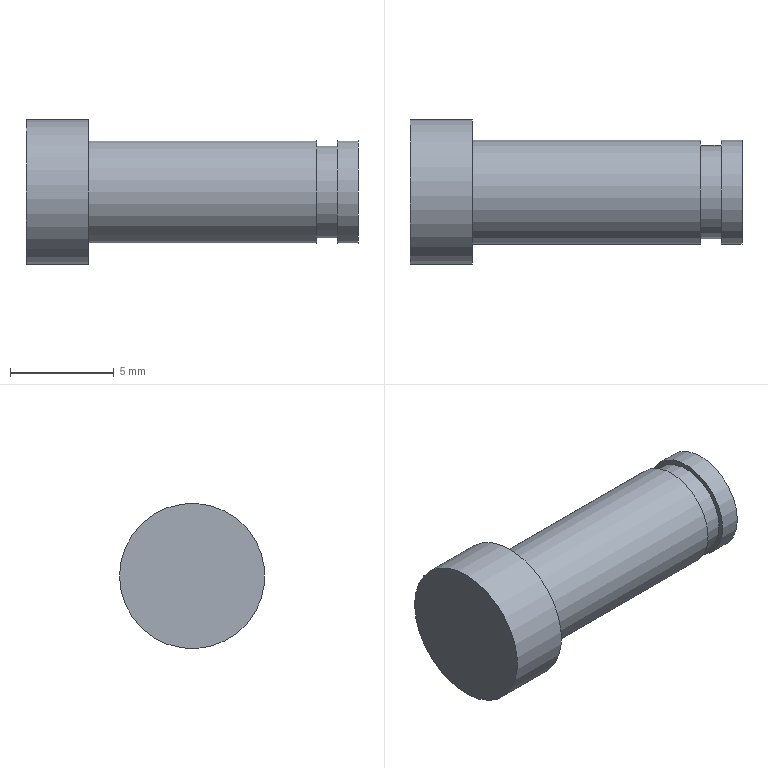Component | NX | PIN | 1 solid | 9 faces | box 16 x 7 x 7 mm | volume 367 mm3 | plane 5 | cylinder 4 | commonest cylinder face diameters 5 x2 7 x1 4.5 x1
STEP:
#1=CARTESIAN_POINT('',(0.,0.,0.));
#2=DIRECTION('',(0.,0.,1.));
#3=DIRECTION('',(1.,0.,0.));
#4=AXIS2_PLACEMENT_3D('',#1,#2,#3);
#5=CARTESIAN_POINT('',(-94.,4.863,83.));
#6=VERTEX_POINT('',#5);
#7=CARTESIAN_POINT('',(-94.,2.363,83.));
#8=DIRECTION('',(1.,0.,0.));
#9=DIRECTION('',(0.,1.,0.));
#10=AXIS2_PLACEMENT_3D('',#7,#8,#9);
#11=CIRCLE('',#10,2.5);
#12=CARTESIAN_POINT('',(-94.,2.363,83.));
#13=DIRECTION('',(1.,0.,0.));
#14=DIRECTION('',(0.,1.,0.));
#15=AXIS2_PLACEMENT_3D('',#12,#13,#14);
#16=PLANE('',#15);
#17=CARTESIAN_POINT('',(0.,0.));
#18=DIRECTION('',(1.,0.));
#19=AXIS2_PLACEMENT_2D('',#17,#18);
#20=CIRCLE('',#19,2.5);
#21=(GEOMETRIC_REPRESENTATION_CONTEXT(2)PARAMETRIC_REPRESENTATION_CONTEXT()REPRESENTATION_CONTEXT('',''));
#22=DEFINITIONAL_REPRESENTATION('',(#20),#21);
#23=PCURVE('',#16,#22);
#24=CARTESIAN_POINT('',(-94.,2.363,83.));
#25=DIRECTION('',(1.,0.,0.));
#26=DIRECTION('',(0.,1.,0.));
#27=AXIS2_PLACEMENT_3D('',#24,#25,#26);
#28=CYLINDRICAL_SURFACE('',#27,2.5);
#29=CARTESIAN_POINT('',(0.,0.));
#30=DIRECTION('',(1.,0.));
#31=VECTOR('',#30,1.);
#32=LINE('',#29,#31);
#33=(GEOMETRIC_REPRESENTATION_CONTEXT(2)PARAMETRIC_REPRESENTATION_CONTEXT()REPRESENTATION_CONTEXT('',''));
#34=DEFINITIONAL_REPRESENTATION('',(#32),#33);
#35=PCURVE('',#28,#34);
#36=SURFACE_CURVE('',#11,(#23,#35),.PCURVE_S1.);
#37=EDGE_CURVE('',#6,#6,#36,.T.);
#38=ORIENTED_EDGE('',*,*,#37,.F.);
#39=EDGE_LOOP('',(#38));
#40=FACE_BOUND('',#39,.T.);
#41=CARTESIAN_POINT('',(-94.,5.863,83.));
#42=VERTEX_POINT('',#41);
#43=CARTESIAN_POINT('',(-94.,2.363,83.));
#44=DIRECTION('',(-1.,0.,0.));
#45=DIRECTION('',(0.,1.,0.));
#46=AXIS2_PLACEMENT_3D('',#43,#44,#45);
#47=CIRCLE('',#46,3.5);
#48=CARTESIAN_POINT('',(3.5,0.));
#49=CARTESIAN_POINT('',(3.5,-6.062));
#50=CARTESIAN_POINT('',(-1.75,-3.031));
#51=CARTESIAN_POINT('',(-7.,-0.));
#52=CARTESIAN_POINT('',(-1.75,3.031));
#53=CARTESIAN_POINT('',(3.5,6.062));
#54=CARTESIAN_POINT('',(3.5,0.));
#55=(BOUNDED_CURVE()B_SPLINE_CURVE(2,(#48,#49,#50,#51,#52,#53,#54),.UNSPECIFIED.,.T.,.F.)B_SPLINE_CURVE_WITH_KNOTS((1,2,2,2,2,1),(-2.094,0.,2.094,4.189,6.283,8.378),.UNSPECIFIED.)CURVE()GEOMETRIC_REPRESENTATION_ITEM()RATIONAL_B_SPLINE_CURVE((1.,0.5,1.,0.5,1.,0.5,1.))REPRESENTATION_ITEM(''));
#56=(GEOMETRIC_REPRESENTATION_CONTEXT(2)PARAMETRIC_REPRESENTATION_CONTEXT()REPRESENTATION_CONTEXT('',''));
#57=DEFINITIONAL_REPRESENTATION('',(#55),#56);
#58=PCURVE('',#16,#57);
#59=CARTESIAN_POINT('',(-97.,2.363,83.));
#60=DIRECTION('',(1.,0.,0.));
#61=DIRECTION('',(0.,1.,0.));
#62=AXIS2_PLACEMENT_3D('',#59,#60,#61);
#63=CYLINDRICAL_SURFACE('',#62,3.5);
#64=CARTESIAN_POINT('',(6.283,3.));
#65=DIRECTION('',(-1.,0.));
#66=VECTOR('',#65,1.);
#67=LINE('',#64,#66);
#68=(GEOMETRIC_REPRESENTATION_CONTEXT(2)PARAMETRIC_REPRESENTATION_CONTEXT()REPRESENTATION_CONTEXT('',''));
#69=DEFINITIONAL_REPRESENTATION('',(#67),#68);
#70=PCURVE('',#63,#69);
#71=SURFACE_CURVE('',#47,(#58,#70),.PCURVE_S1.);
#72=EDGE_CURVE('',#42,#42,#71,.T.);
#73=ORIENTED_EDGE('',*,*,#72,.F.);
#74=EDGE_LOOP('',(#73));
#75=FACE_BOUND('',#74,.T.);
#76=ADVANCED_FACE('',(#40,#75),#16,.T.);
#77=CARTESIAN_POINT('',(-97.,5.863,83.));
#78=VERTEX_POINT('',#77);
#79=CARTESIAN_POINT('',(-97.,2.363,83.));
#80=DIRECTION('',(1.,0.,0.));
#81=DIRECTION('',(0.,1.,0.));
#82=AXIS2_PLACEMENT_3D('',#79,#80,#81);
#83=CIRCLE('',#82,3.5);
#84=CARTESIAN_POINT('',(-97.,2.363,83.));
#85=DIRECTION('',(-1.,0.,0.));
#86=DIRECTION('',(0.,-1.,0.));
#87=AXIS2_PLACEMENT_3D('',#84,#85,#86);
#88=PLANE('',#87);
#89=CARTESIAN_POINT('',(-3.5,0.));
#90=CARTESIAN_POINT('',(-3.5,6.062));
#91=CARTESIAN_POINT('',(1.75,3.031));
#92=CARTESIAN_POINT('',(7.,0.));
#93=CARTESIAN_POINT('',(1.75,-3.031));
#94=CARTESIAN_POINT('',(-3.5,-6.062));
#95=CARTESIAN_POINT('',(-3.5,0.));
#96=(BOUNDED_CURVE()B_SPLINE_CURVE(2,(#89,#90,#91,#92,#93,#94,#95),.UNSPECIFIED.,.T.,.F.)B_SPLINE_CURVE_WITH_KNOTS((1,2,2,2,2,1),(-2.094,0.,2.094,4.189,6.283,8.378),.UNSPECIFIED.)CURVE()GEOMETRIC_REPRESENTATION_ITEM()RATIONAL_B_SPLINE_CURVE((1.,0.5,1.,0.5,1.,0.5,1.))REPRESENTATION_ITEM(''));
#97=(GEOMETRIC_REPRESENTATION_CONTEXT(2)PARAMETRIC_REPRESENTATION_CONTEXT()REPRESENTATION_CONTEXT('',''));
#98=DEFINITIONAL_REPRESENTATION('',(#96),#97);
#99=PCURVE('',#88,#98);
#100=CARTESIAN_POINT('',(0.,0.));
#101=DIRECTION('',(1.,0.));
#102=VECTOR('',#101,1.);
#103=LINE('',#100,#102);
#104=(GEOMETRIC_REPRESENTATION_CONTEXT(2)PARAMETRIC_REPRESENTATION_CONTEXT()REPRESENTATION_CONTEXT('',''));
#105=DEFINITIONAL_REPRESENTATION('',(#103),#104);
#106=PCURVE('',#63,#105);
#107=SURFACE_CURVE('',#83,(#99,#106),.PCURVE_S1.);
#108=EDGE_CURVE('',#78,#78,#107,.T.);
#109=ORIENTED_EDGE('',*,*,#108,.F.);
#110=EDGE_LOOP('',(#109));
#111=FACE_BOUND('',#110,.T.);
#112=ADVANCED_FACE('',(#111),#88,.T.);
#113=ORIENTED_EDGE('',*,*,#72,.T.);
#114=CARTESIAN_POINT('',(-97.,5.863,83.));
#115=CARTESIAN_POINT('',(-94.,5.863,83.));
#116=B_SPLINE_CURVE_WITH_KNOTS('',1,(#114,#115),.UNSPECIFIED.,.F.,.F.,(2,2),(0.,3.),.PIECEWISE_BEZIER_KNOTS.);
#117=CARTESIAN_POINT('',(0.,0.));
#118=DIRECTION('',(0.,1.));
#119=VECTOR('',#118,1.);
#120=LINE('',#117,#119);
#121=(GEOMETRIC_REPRESENTATION_CONTEXT(2)PARAMETRIC_REPRESENTATION_CONTEXT()REPRESENTATION_CONTEXT('',''));
#122=DEFINITIONAL_REPRESENTATION('',(#120),#121);
#123=PCURVE('',#63,#122);
#124=CARTESIAN_POINT('',(6.283,0.));
#125=DIRECTION('',(0.,1.));
#126=VECTOR('',#125,1.);
#127=LINE('',#124,#126);
#128=(GEOMETRIC_REPRESENTATION_CONTEXT(2)PARAMETRIC_REPRESENTATION_CONTEXT()REPRESENTATION_CONTEXT('',''));
#129=DEFINITIONAL_REPRESENTATION('',(#127),#128);
#130=PCURVE('',#63,#129);
#131=SEAM_CURVE('',#116,(#123,#130),.PCURVE_S1.);
#132=EDGE_CURVE('',#78,#42,#131,.T.);
#133=ORIENTED_EDGE('',*,*,#132,.F.);
#134=ORIENTED_EDGE('',*,*,#108,.T.);
#135=ORIENTED_EDGE('',*,*,#132,.T.);
#136=EDGE_LOOP('',(#113,#133,#134,#135));
#137=FACE_BOUND('',#136,.T.);
#138=ADVANCED_FACE('',(#137),#63,.T.);
#139=CARTESIAN_POINT('',(-83.,4.613,83.));
#140=VERTEX_POINT('',#139);
#141=CARTESIAN_POINT('',(-83.,2.363,83.));
#142=DIRECTION('',(1.,0.,0.));
#143=DIRECTION('',(0.,1.,0.));
#144=AXIS2_PLACEMENT_3D('',#141,#142,#143);
#145=CIRCLE('',#144,2.25);
#146=CARTESIAN_POINT('',(-83.,2.363,83.));
#147=DIRECTION('',(1.,0.,0.));
#148=DIRECTION('',(0.,1.,0.));
#149=AXIS2_PLACEMENT_3D('',#146,#147,#148);
#150=PLANE('',#149);
#151=CARTESIAN_POINT('',(0.,0.));
#152=DIRECTION('',(1.,0.));
#153=AXIS2_PLACEMENT_2D('',#151,#152);
#154=CIRCLE('',#153,2.25);
#155=(GEOMETRIC_REPRESENTATION_CONTEXT(2)PARAMETRIC_REPRESENTATION_CONTEXT()REPRESENTATION_CONTEXT('',''));
#156=DEFINITIONAL_REPRESENTATION('',(#154),#155);
#157=PCURVE('',#150,#156);
#158=CARTESIAN_POINT('',(-83.,2.363,83.));
#159=DIRECTION('',(1.,0.,0.));
#160=DIRECTION('',(0.,1.,0.));
#161=AXIS2_PLACEMENT_3D('',#158,#159,#160);
#162=CYLINDRICAL_SURFACE('',#161,2.25);
#163=CARTESIAN_POINT('',(0.,0.));
#164=DIRECTION('',(1.,0.));
#165=VECTOR('',#164,1.);
#166=LINE('',#163,#165);
#167=(GEOMETRIC_REPRESENTATION_CONTEXT(2)PARAMETRIC_REPRESENTATION_CONTEXT()REPRESENTATION_CONTEXT('',''));
#168=DEFINITIONAL_REPRESENTATION('',(#166),#167);
#169=PCURVE('',#162,#168);
#170=SURFACE_CURVE('',#145,(#157,#169),.PCURVE_S1.);
#171=EDGE_CURVE('',#140,#140,#170,.T.);
#172=ORIENTED_EDGE('',*,*,#171,.F.);
#173=EDGE_LOOP('',(#172));
#174=FACE_BOUND('',#173,.T.);
#175=CARTESIAN_POINT('',(-83.,4.863,83.));
#176=VERTEX_POINT('',#175);
#177=CARTESIAN_POINT('',(-83.,2.363,83.));
#178=DIRECTION('',(1.,0.,0.));
#179=DIRECTION('',(0.,1.,0.));
#180=AXIS2_PLACEMENT_3D('',#177,#178,#179);
#181=CIRCLE('',#180,2.5);
#182=CARTESIAN_POINT('',(0.,0.));
#183=DIRECTION('',(1.,0.));
#184=AXIS2_PLACEMENT_2D('',#182,#183);
#185=CIRCLE('',#184,2.5);
#186=(GEOMETRIC_REPRESENTATION_CONTEXT(2)PARAMETRIC_REPRESENTATION_CONTEXT()REPRESENTATION_CONTEXT('',''));
#187=DEFINITIONAL_REPRESENTATION('',(#185),#186);
#188=PCURVE('',#150,#187);
#189=CARTESIAN_POINT('',(0.,11.));
#190=DIRECTION('',(1.,0.));
#191=VECTOR('',#190,1.);
#192=LINE('',#189,#191);
#193=(GEOMETRIC_REPRESENTATION_CONTEXT(2)PARAMETRIC_REPRESENTATION_CONTEXT()REPRESENTATION_CONTEXT('',''));
#194=DEFINITIONAL_REPRESENTATION('',(#192),#193);
#195=PCURVE('',#28,#194);
#196=SURFACE_CURVE('',#181,(#188,#195),.PCURVE_S1.);
#197=EDGE_CURVE('',#176,#176,#196,.T.);
#198=ORIENTED_EDGE('',*,*,#197,.T.);
#199=EDGE_LOOP('',(#198));
#200=FACE_BOUND('',#199,.T.);
#201=ADVANCED_FACE('',(#174,#200),#150,.T.);
#202=ORIENTED_EDGE('',*,*,#197,.F.);
#203=CARTESIAN_POINT('',(-94.,4.863,83.));
#204=CARTESIAN_POINT('',(-83.,4.863,83.));
#205=B_SPLINE_CURVE_WITH_KNOTS('',1,(#203,#204),.UNSPECIFIED.,.F.,.F.,(2,2),(0.,11.),.PIECEWISE_BEZIER_KNOTS.);
#206=CARTESIAN_POINT('',(0.,0.));
#207=DIRECTION('',(0.,1.));
#208=VECTOR('',#207,1.);
#209=LINE('',#206,#208);
#210=(GEOMETRIC_REPRESENTATION_CONTEXT(2)PARAMETRIC_REPRESENTATION_CONTEXT()REPRESENTATION_CONTEXT('',''));
#211=DEFINITIONAL_REPRESENTATION('',(#209),#210);
#212=PCURVE('',#28,#211);
#213=CARTESIAN_POINT('',(6.283,0.));
#214=DIRECTION('',(0.,1.));
#215=VECTOR('',#214,1.);
#216=LINE('',#213,#215);
#217=(GEOMETRIC_REPRESENTATION_CONTEXT(2)PARAMETRIC_REPRESENTATION_CONTEXT()REPRESENTATION_CONTEXT('',''));
#218=DEFINITIONAL_REPRESENTATION('',(#216),#217);
#219=PCURVE('',#28,#218);
#220=SEAM_CURVE('',#205,(#212,#219),.PCURVE_S1.);
#221=EDGE_CURVE('',#6,#176,#220,.T.);
#222=ORIENTED_EDGE('',*,*,#221,.F.);
#223=ORIENTED_EDGE('',*,*,#37,.T.);
#224=ORIENTED_EDGE('',*,*,#221,.T.);
#225=EDGE_LOOP('',(#202,#222,#223,#224));
#226=FACE_BOUND('',#225,.T.);
#227=ADVANCED_FACE('',(#226),#28,.T.);
#228=CARTESIAN_POINT('',(-82.,4.613,83.));
#229=VERTEX_POINT('',#228);
#230=CARTESIAN_POINT('',(-82.,2.363,83.));
#231=DIRECTION('',(1.,0.,0.));
#232=DIRECTION('',(0.,1.,0.));
#233=AXIS2_PLACEMENT_3D('',#230,#231,#232);
#234=CIRCLE('',#233,2.25);
#235=CARTESIAN_POINT('',(0.,1.));
#236=DIRECTION('',(1.,0.));
#237=VECTOR('',#236,1.);
#238=LINE('',#235,#237);
#239=(GEOMETRIC_REPRESENTATION_CONTEXT(2)PARAMETRIC_REPRESENTATION_CONTEXT()REPRESENTATION_CONTEXT('',''));
#240=DEFINITIONAL_REPRESENTATION('',(#238),#239);
#241=PCURVE('',#162,#240);
#242=CARTESIAN_POINT('',(-82.,2.363,83.));
#243=DIRECTION('',(-1.,0.,0.));
#244=DIRECTION('',(0.,-1.,0.));
#245=AXIS2_PLACEMENT_3D('',#242,#243,#244);
#246=PLANE('',#245);
#247=CARTESIAN_POINT('',(-2.25,0.));
#248=CARTESIAN_POINT('',(-2.25,3.897));
#249=CARTESIAN_POINT('',(1.125,1.949));
#250=CARTESIAN_POINT('',(4.5,0.));
#251=CARTESIAN_POINT('',(1.125,-1.949));
#252=CARTESIAN_POINT('',(-2.25,-3.897));
#253=CARTESIAN_POINT('',(-2.25,0.));
#254=(BOUNDED_CURVE()B_SPLINE_CURVE(2,(#247,#248,#249,#250,#251,#252,#253),.UNSPECIFIED.,.T.,.F.)B_SPLINE_CURVE_WITH_KNOTS((1,2,2,2,2,1),(-2.094,0.,2.094,4.189,6.283,8.378),.UNSPECIFIED.)CURVE()GEOMETRIC_REPRESENTATION_ITEM()RATIONAL_B_SPLINE_CURVE((1.,0.5,1.,0.5,1.,0.5,1.))REPRESENTATION_ITEM(''));
#255=(GEOMETRIC_REPRESENTATION_CONTEXT(2)PARAMETRIC_REPRESENTATION_CONTEXT()REPRESENTATION_CONTEXT('',''));
#256=DEFINITIONAL_REPRESENTATION('',(#254),#255);
#257=PCURVE('',#246,#256);
#258=SURFACE_CURVE('',#234,(#241,#257),.PCURVE_S1.);
#259=EDGE_CURVE('',#229,#229,#258,.T.);
#260=ORIENTED_EDGE('',*,*,#259,.F.);
#261=CARTESIAN_POINT('',(-83.,4.613,83.));
#262=CARTESIAN_POINT('',(-82.,4.613,83.));
#263=B_SPLINE_CURVE_WITH_KNOTS('',1,(#261,#262),.UNSPECIFIED.,.F.,.F.,(2,2),(0.,1.),.PIECEWISE_BEZIER_KNOTS.);
#264=CARTESIAN_POINT('',(0.,0.));
#265=DIRECTION('',(0.,1.));
#266=VECTOR('',#265,1.);
#267=LINE('',#264,#266);
#268=(GEOMETRIC_REPRESENTATION_CONTEXT(2)PARAMETRIC_REPRESENTATION_CONTEXT()REPRESENTATION_CONTEXT('',''));
#269=DEFINITIONAL_REPRESENTATION('',(#267),#268);
#270=PCURVE('',#162,#269);
#271=CARTESIAN_POINT('',(6.283,0.));
#272=DIRECTION('',(0.,1.));
#273=VECTOR('',#272,1.);
#274=LINE('',#271,#273);
#275=(GEOMETRIC_REPRESENTATION_CONTEXT(2)PARAMETRIC_REPRESENTATION_CONTEXT()REPRESENTATION_CONTEXT('',''));
#276=DEFINITIONAL_REPRESENTATION('',(#274),#275);
#277=PCURVE('',#162,#276);
#278=SEAM_CURVE('',#263,(#270,#277),.PCURVE_S1.);
#279=EDGE_CURVE('',#140,#229,#278,.T.);
#280=ORIENTED_EDGE('',*,*,#279,.F.);
#281=ORIENTED_EDGE('',*,*,#171,.T.);
#282=ORIENTED_EDGE('',*,*,#279,.T.);
#283=EDGE_LOOP('',(#260,#280,#281,#282));
#284=FACE_BOUND('',#283,.T.);
#285=ADVANCED_FACE('',(#284),#162,.T.);
#286=CARTESIAN_POINT('',(-81.,4.863,83.));
#287=VERTEX_POINT('',#286);
#288=CARTESIAN_POINT('',(-81.,2.363,83.));
#289=DIRECTION('',(1.,0.,0.));
#290=DIRECTION('',(0.,1.,0.));
#291=AXIS2_PLACEMENT_3D('',#288,#289,#290);
#292=CIRCLE('',#291,2.5);
#293=CARTESIAN_POINT('',(-81.,2.363,83.));
#294=DIRECTION('',(1.,0.,0.));
#295=DIRECTION('',(0.,1.,0.));
#296=AXIS2_PLACEMENT_3D('',#293,#294,#295);
#297=PLANE('',#296);
#298=CARTESIAN_POINT('',(0.,0.));
#299=DIRECTION('',(1.,0.));
#300=AXIS2_PLACEMENT_2D('',#298,#299);
#301=CIRCLE('',#300,2.5);
#302=(GEOMETRIC_REPRESENTATION_CONTEXT(2)PARAMETRIC_REPRESENTATION_CONTEXT()REPRESENTATION_CONTEXT('',''));
#303=DEFINITIONAL_REPRESENTATION('',(#301),#302);
#304=PCURVE('',#297,#303);
#305=CARTESIAN_POINT('',(-82.,2.363,83.));
#306=DIRECTION('',(1.,0.,0.));
#307=DIRECTION('',(0.,1.,0.));
#308=AXIS2_PLACEMENT_3D('',#305,#306,#307);
#309=CYLINDRICAL_SURFACE('',#308,2.5);
#310=CARTESIAN_POINT('',(0.,1.));
#311=DIRECTION('',(1.,0.));
#312=VECTOR('',#311,1.);
#313=LINE('',#310,#312);
#314=(GEOMETRIC_REPRESENTATION_CONTEXT(2)PARAMETRIC_REPRESENTATION_CONTEXT()REPRESENTATION_CONTEXT('',''));
#315=DEFINITIONAL_REPRESENTATION('',(#313),#314);
#316=PCURVE('',#309,#315);
#317=SURFACE_CURVE('',#292,(#304,#316),.PCURVE_S1.);
#318=EDGE_CURVE('',#287,#287,#317,.T.);
#319=ORIENTED_EDGE('',*,*,#318,.T.);
#320=EDGE_LOOP('',(#319));
#321=FACE_BOUND('',#320,.T.);
#322=ADVANCED_FACE('',(#321),#297,.T.);
#323=ORIENTED_EDGE('',*,*,#259,.T.);
#324=EDGE_LOOP('',(#323));
#325=FACE_BOUND('',#324,.T.);
#326=CARTESIAN_POINT('',(-82.,4.863,83.));
#327=VERTEX_POINT('',#326);
#328=CARTESIAN_POINT('',(-82.,2.363,83.));
#329=DIRECTION('',(1.,0.,0.));
#330=DIRECTION('',(0.,1.,0.));
#331=AXIS2_PLACEMENT_3D('',#328,#329,#330);
#332=CIRCLE('',#331,2.5);
#333=CARTESIAN_POINT('',(-2.5,0.));
#334=CARTESIAN_POINT('',(-2.5,4.33));
#335=CARTESIAN_POINT('',(1.25,2.165));
#336=CARTESIAN_POINT('',(5.,0.));
#337=CARTESIAN_POINT('',(1.25,-2.165));
#338=CARTESIAN_POINT('',(-2.5,-4.33));
#339=CARTESIAN_POINT('',(-2.5,0.));
#340=(BOUNDED_CURVE()B_SPLINE_CURVE(2,(#333,#334,#335,#336,#337,#338,#339),.UNSPECIFIED.,.T.,.F.)B_SPLINE_CURVE_WITH_KNOTS((1,2,2,2,2,1),(-2.094,0.,2.094,4.189,6.283,8.378),.UNSPECIFIED.)CURVE()GEOMETRIC_REPRESENTATION_ITEM()RATIONAL_B_SPLINE_CURVE((1.,0.5,1.,0.5,1.,0.5,1.))REPRESENTATION_ITEM(''));
#341=(GEOMETRIC_REPRESENTATION_CONTEXT(2)PARAMETRIC_REPRESENTATION_CONTEXT()REPRESENTATION_CONTEXT('',''));
#342=DEFINITIONAL_REPRESENTATION('',(#340),#341);
#343=PCURVE('',#246,#342);
#344=CARTESIAN_POINT('',(0.,0.));
#345=DIRECTION('',(1.,0.));
#346=VECTOR('',#345,1.);
#347=LINE('',#344,#346);
#348=(GEOMETRIC_REPRESENTATION_CONTEXT(2)PARAMETRIC_REPRESENTATION_CONTEXT()REPRESENTATION_CONTEXT('',''));
#349=DEFINITIONAL_REPRESENTATION('',(#347),#348);
#350=PCURVE('',#309,#349);
#351=SURFACE_CURVE('',#332,(#343,#350),.PCURVE_S1.);
#352=EDGE_CURVE('',#327,#327,#351,.T.);
#353=ORIENTED_EDGE('',*,*,#352,.F.);
#354=EDGE_LOOP('',(#353));
#355=FACE_BOUND('',#354,.T.);
#356=ADVANCED_FACE('',(#325,#355),#246,.T.);
#357=ORIENTED_EDGE('',*,*,#318,.F.);
#358=CARTESIAN_POINT('',(-82.,4.863,83.));
#359=CARTESIAN_POINT('',(-81.,4.863,83.));
#360=B_SPLINE_CURVE_WITH_KNOTS('',1,(#358,#359),.UNSPECIFIED.,.F.,.F.,(2,2),(0.,1.),.PIECEWISE_BEZIER_KNOTS.);
#361=CARTESIAN_POINT('',(0.,0.));
#362=DIRECTION('',(0.,1.));
#363=VECTOR('',#362,1.);
#364=LINE('',#361,#363);
#365=(GEOMETRIC_REPRESENTATION_CONTEXT(2)PARAMETRIC_REPRESENTATION_CONTEXT()REPRESENTATION_CONTEXT('',''));
#366=DEFINITIONAL_REPRESENTATION('',(#364),#365);
#367=PCURVE('',#309,#366);
#368=CARTESIAN_POINT('',(6.283,0.));
#369=DIRECTION('',(0.,1.));
#370=VECTOR('',#369,1.);
#371=LINE('',#368,#370);
#372=(GEOMETRIC_REPRESENTATION_CONTEXT(2)PARAMETRIC_REPRESENTATION_CONTEXT()REPRESENTATION_CONTEXT('',''));
#373=DEFINITIONAL_REPRESENTATION('',(#371),#372);
#374=PCURVE('',#309,#373);
#375=SEAM_CURVE('',#360,(#367,#374),.PCURVE_S1.);
#376=EDGE_CURVE('',#327,#287,#375,.T.);
#377=ORIENTED_EDGE('',*,*,#376,.F.);
#378=ORIENTED_EDGE('',*,*,#352,.T.);
#379=ORIENTED_EDGE('',*,*,#376,.T.);
#380=EDGE_LOOP('',(#357,#377,#378,#379));
#381=FACE_BOUND('',#380,.T.);
#382=ADVANCED_FACE('',(#381),#309,.T.);
#383=CLOSED_SHELL('',(#76,#112,#138,#201,#227,#285,#322,#356,#382));
#384=MANIFOLD_SOLID_BREP('',#383);
#385=(LENGTH_UNIT()NAMED_UNIT(*)SI_UNIT(.MILLI.,.METRE.));
#386=UNCERTAINTY_MEASURE_WITH_UNIT(LENGTH_MEASURE(0.00001),#385,'','');
#387=(NAMED_UNIT(*)PLANE_ANGLE_UNIT()SI_UNIT($,.RADIAN.));
#388=(NAMED_UNIT(*)SI_UNIT($,.STERADIAN.)SOLID_ANGLE_UNIT());
#389=(GEOMETRIC_REPRESENTATION_CONTEXT(3)GLOBAL_UNCERTAINTY_ASSIGNED_CONTEXT((#386))GLOBAL_UNIT_ASSIGNED_CONTEXT((#385,#387,#388))REPRESENTATION_CONTEXT('',''));
#390=ADVANCED_BREP_SHAPE_REPRESENTATION('',(#4,#384),#389);